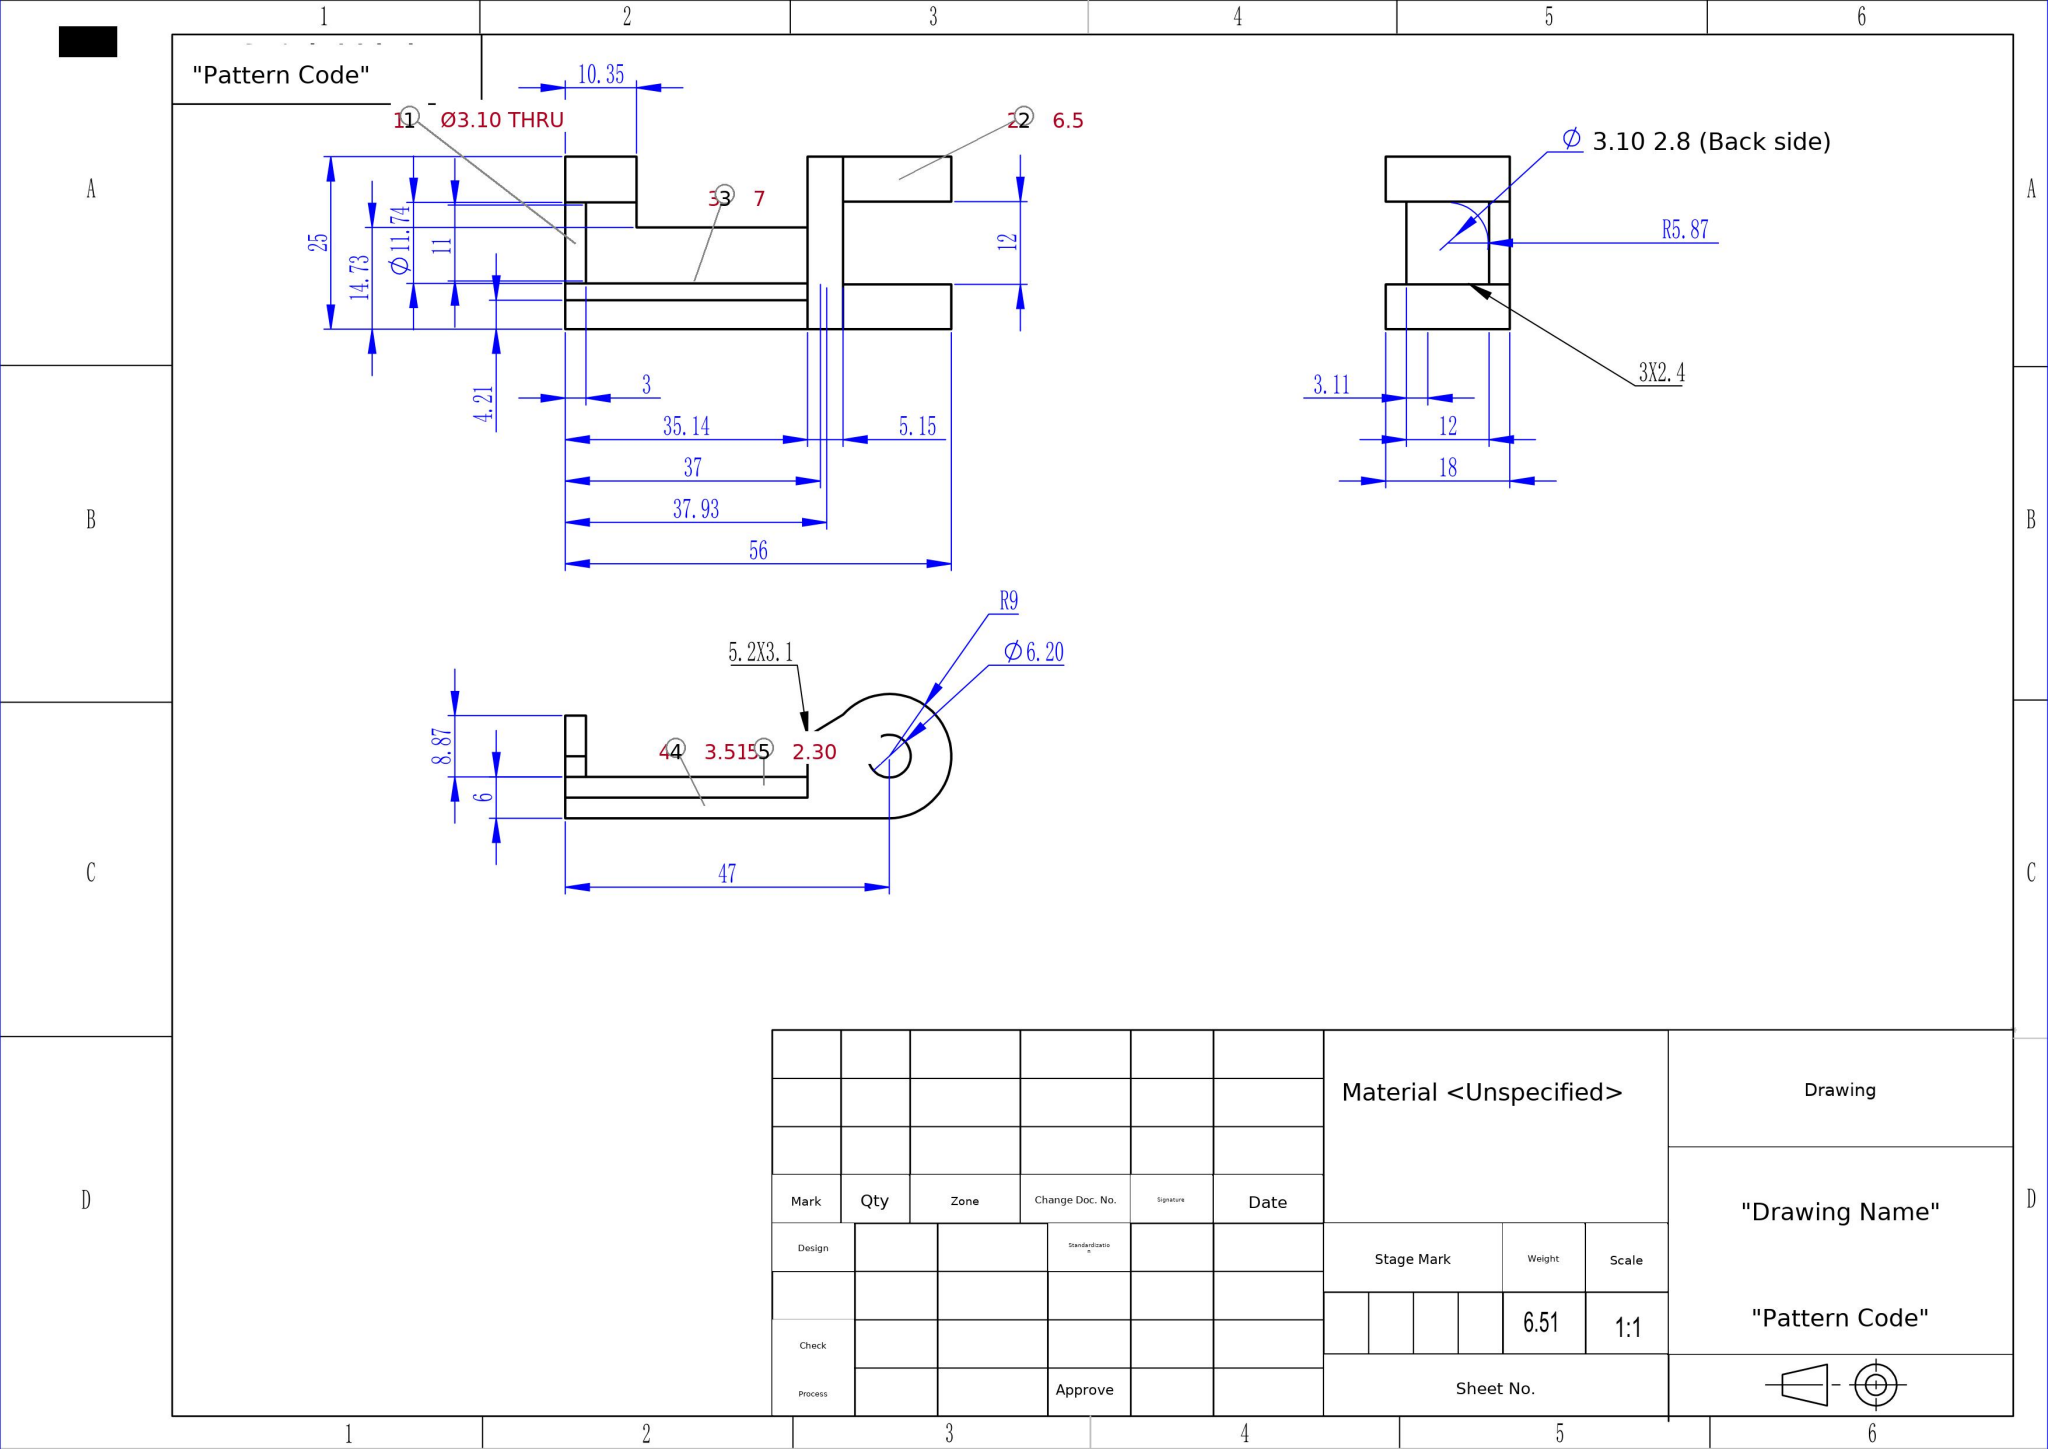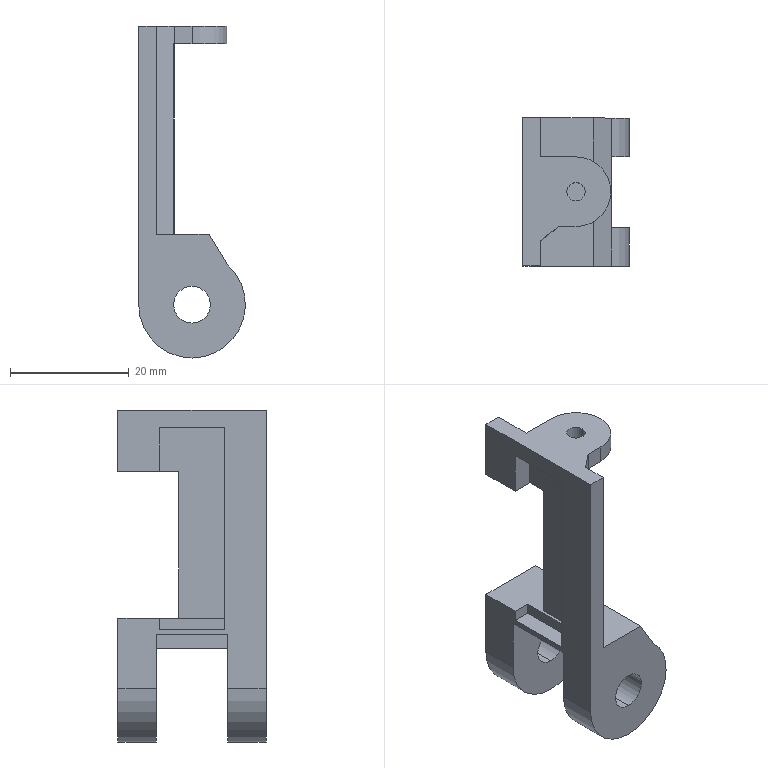Part | SolidWorks | mm | 1 solid | 44 faces | box 18 x 25 x 56 mm | volume 6514 mm3 | plane 30 | cylinder 14 | commonest cylinder face diameters 3.1 x4 6.2 x4 18 x4 11.743 x2